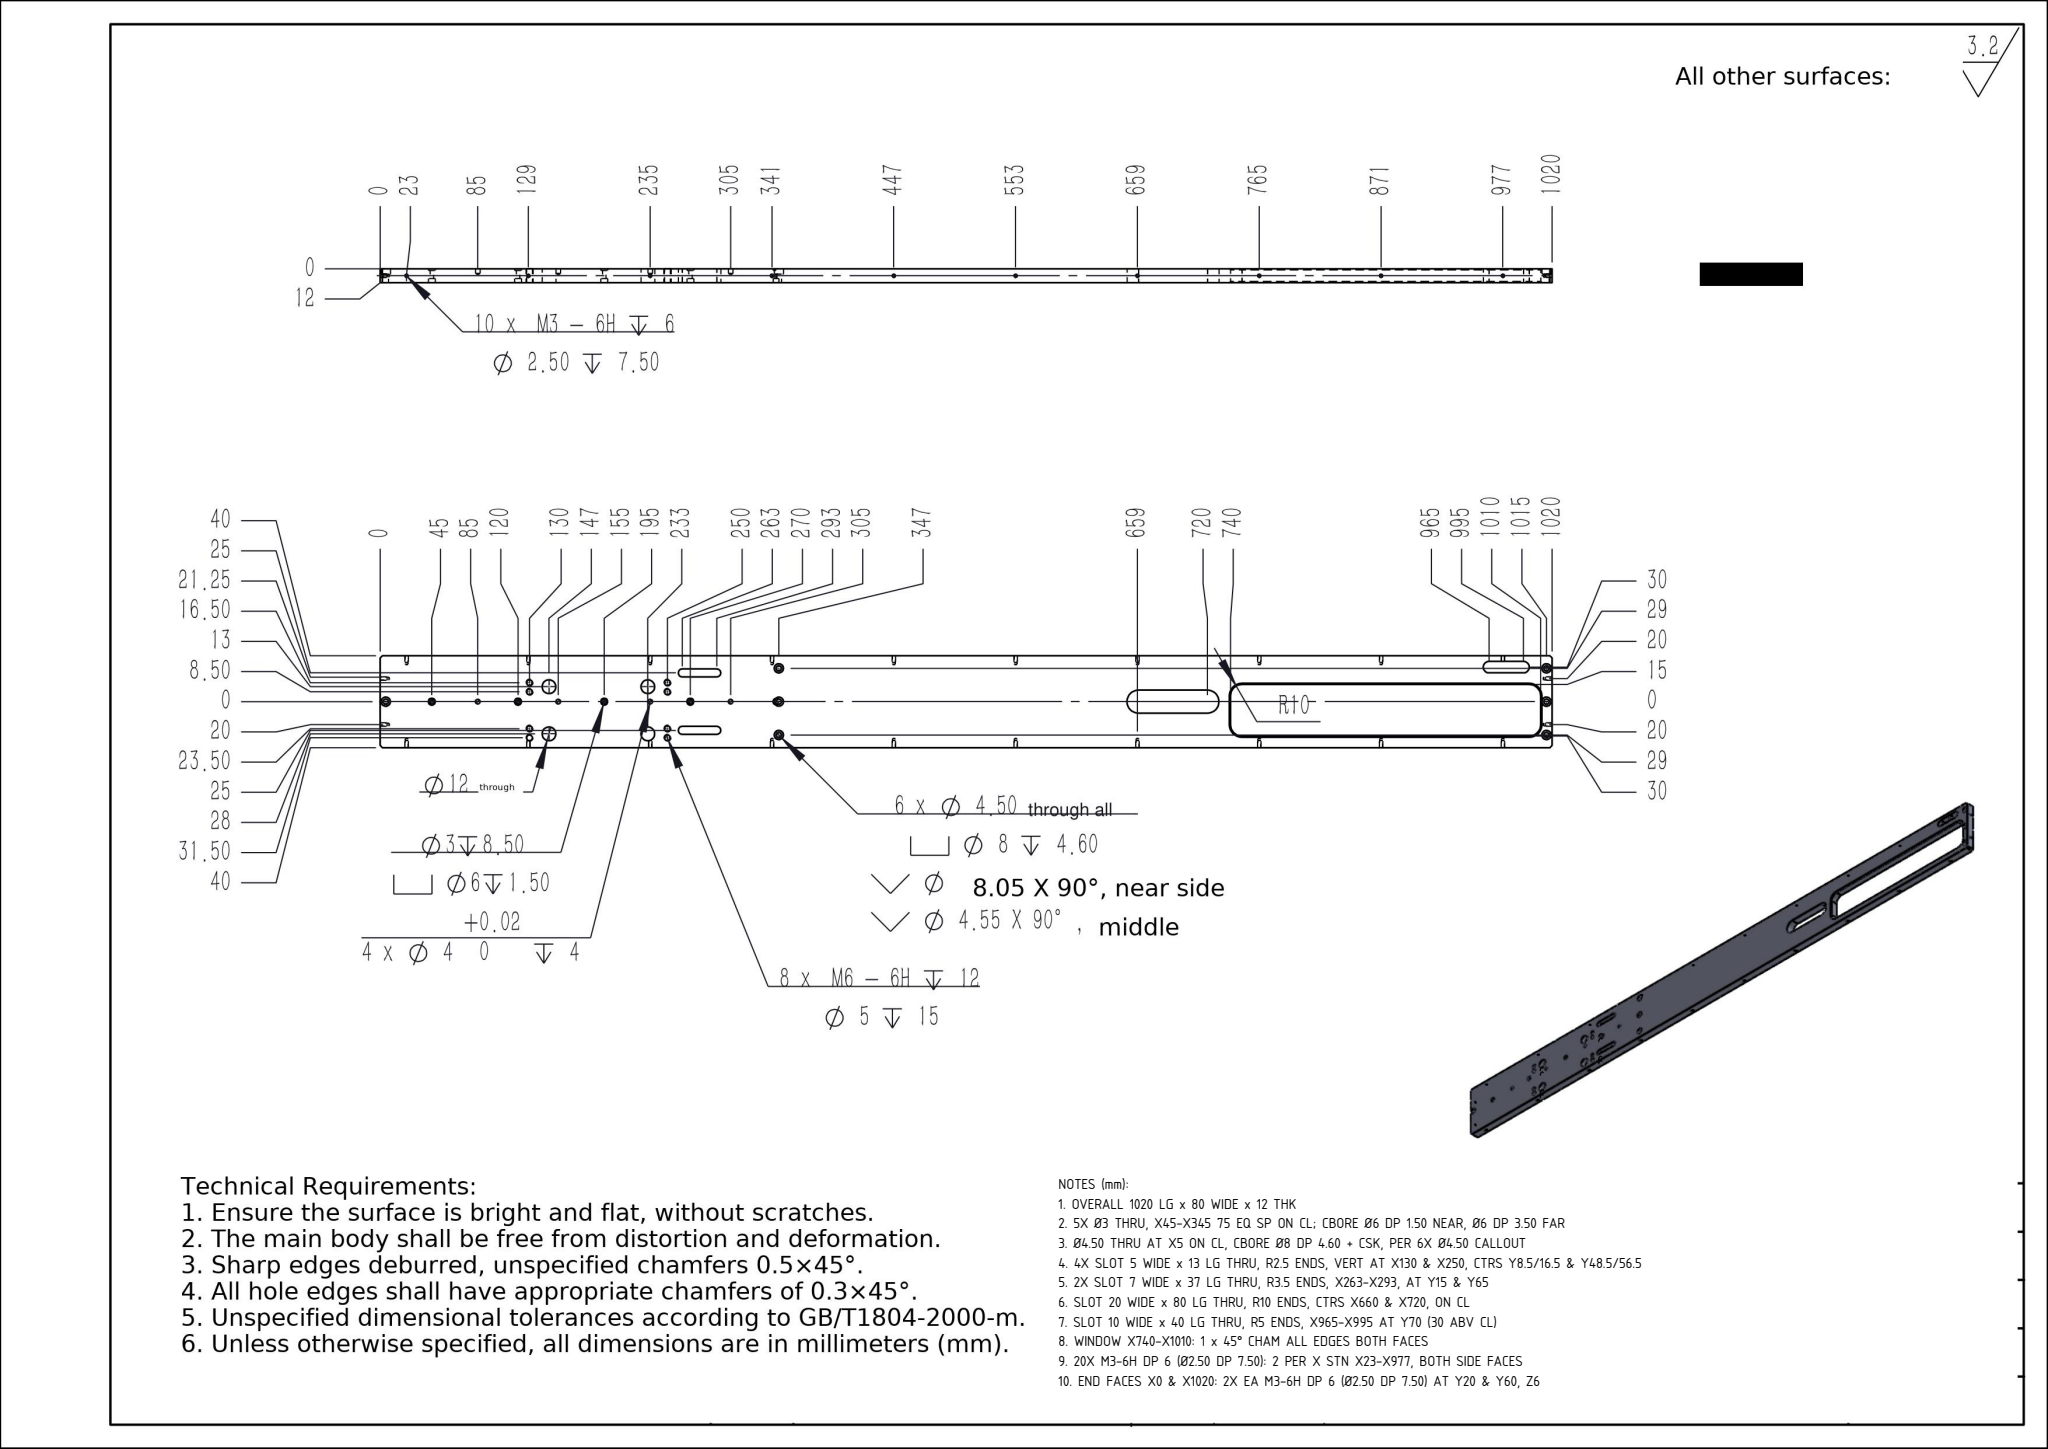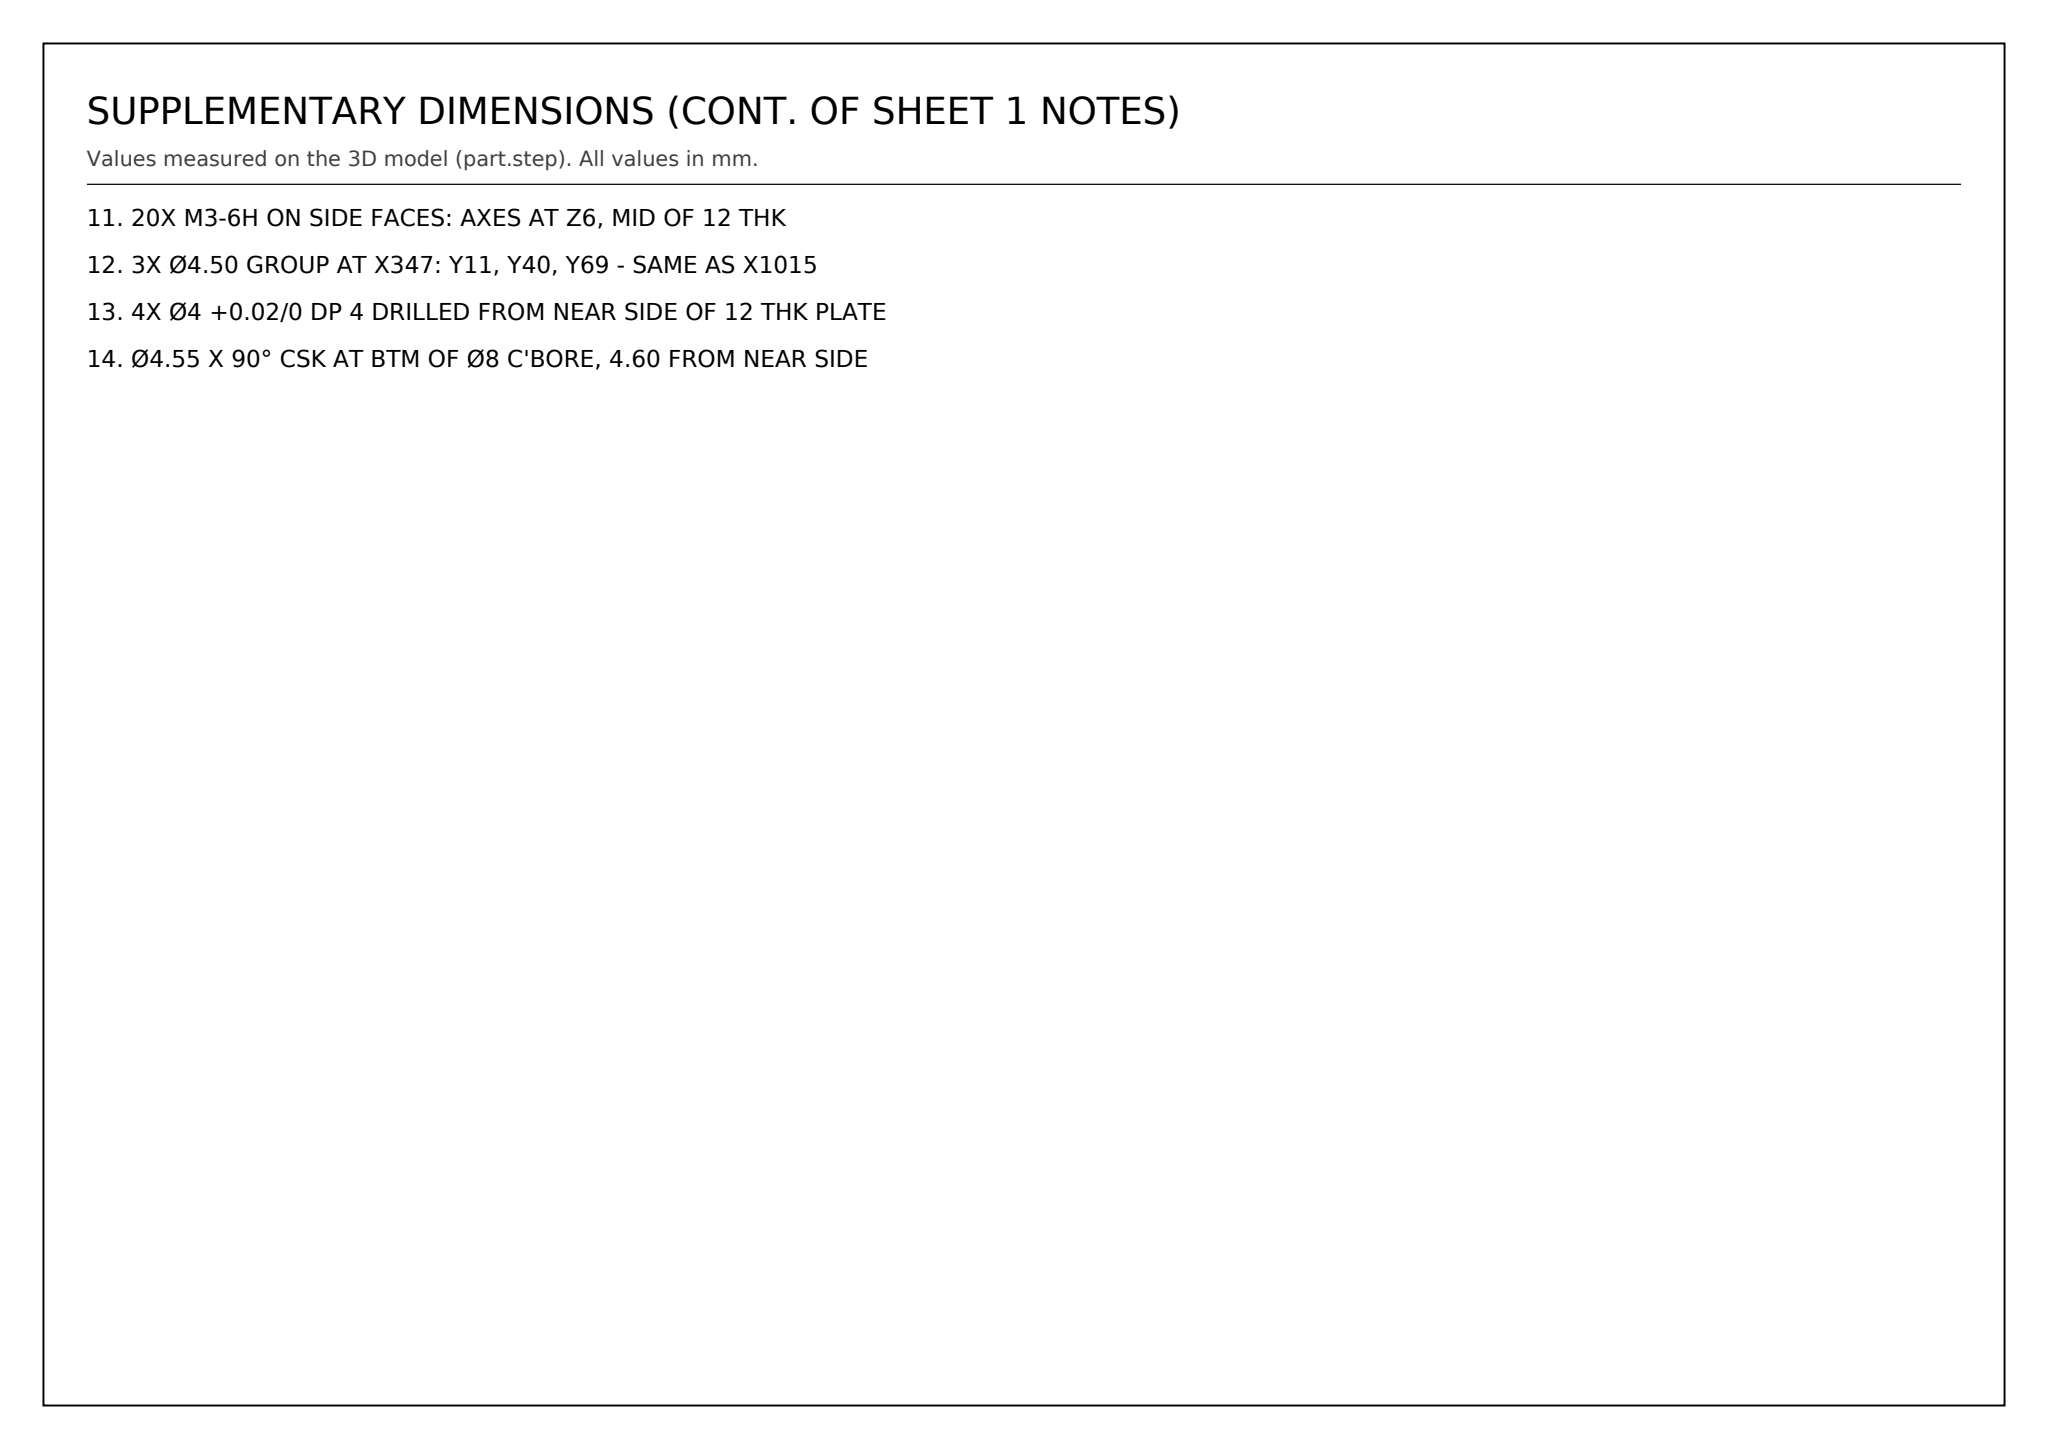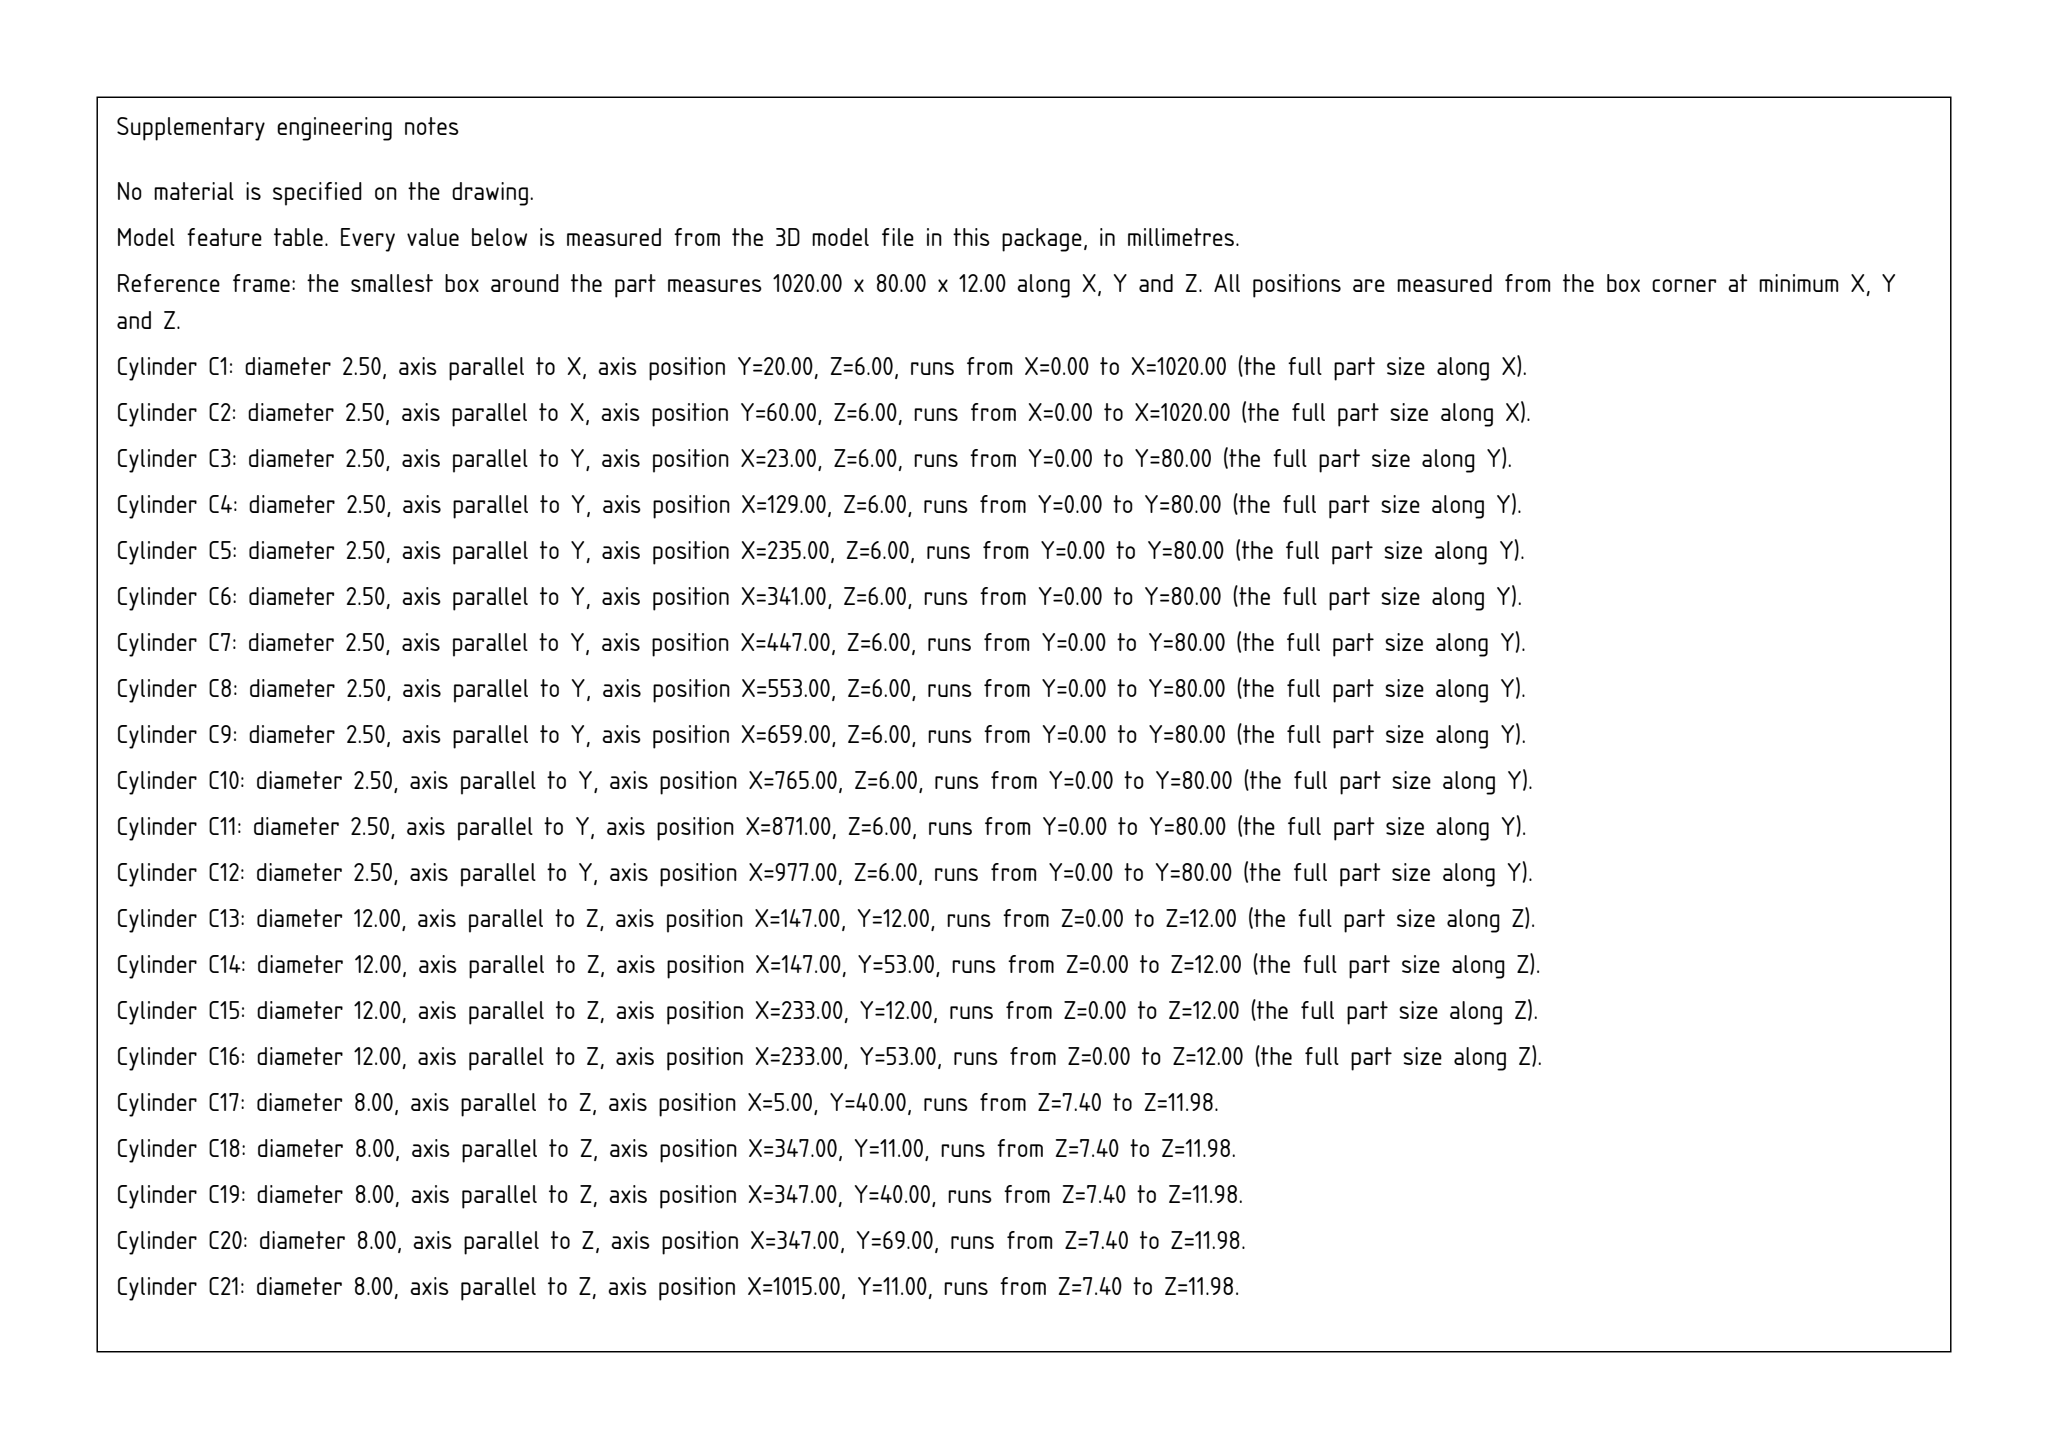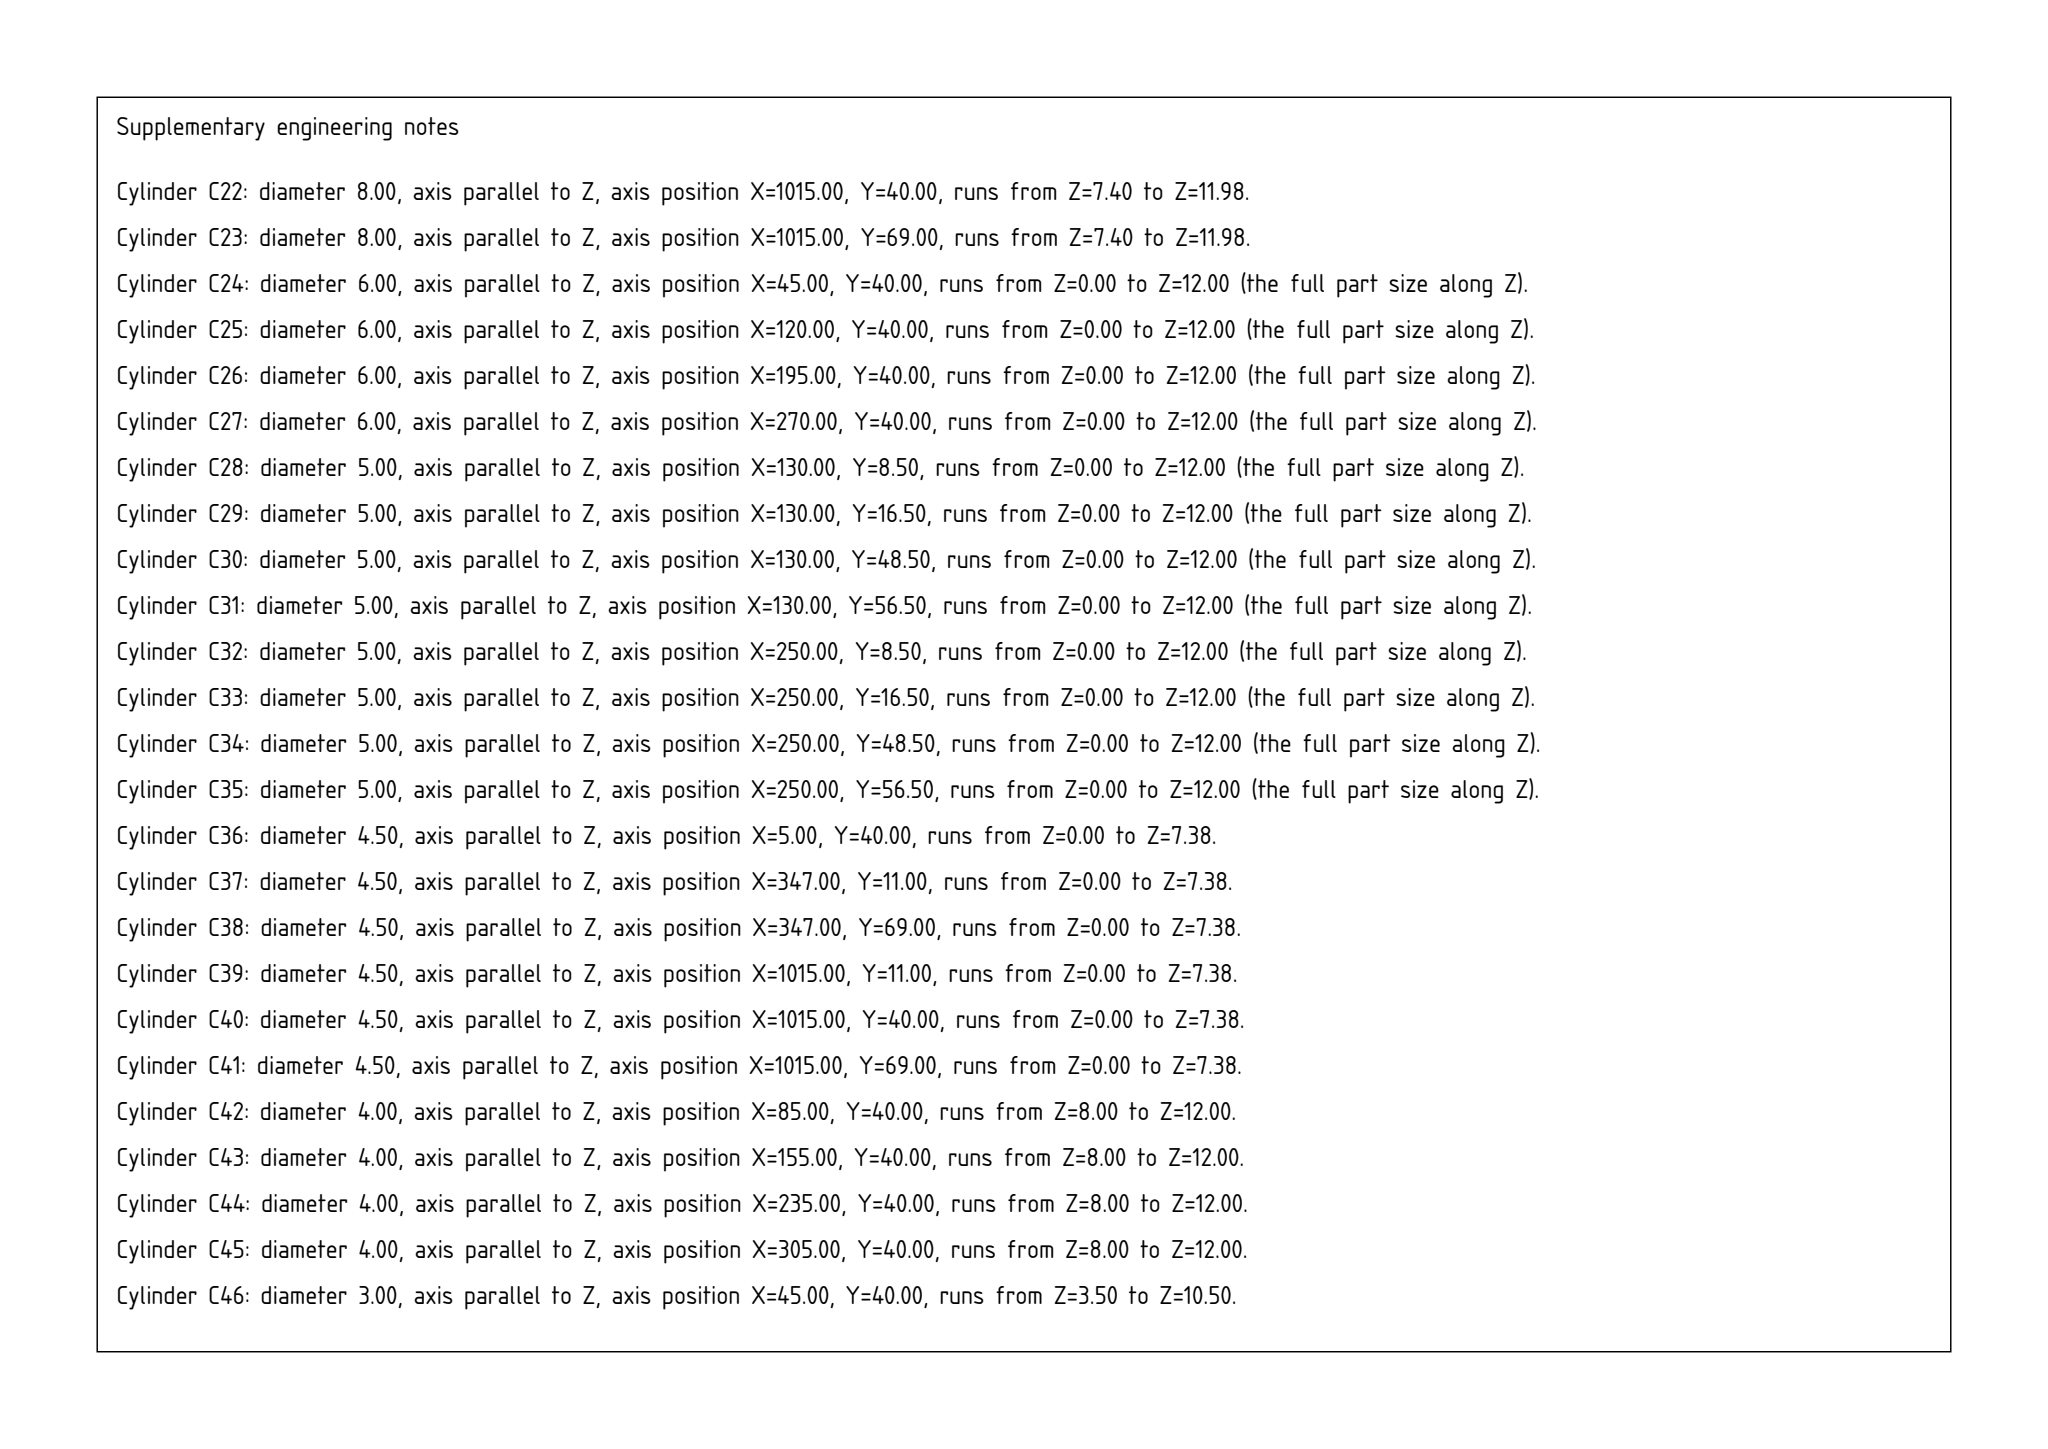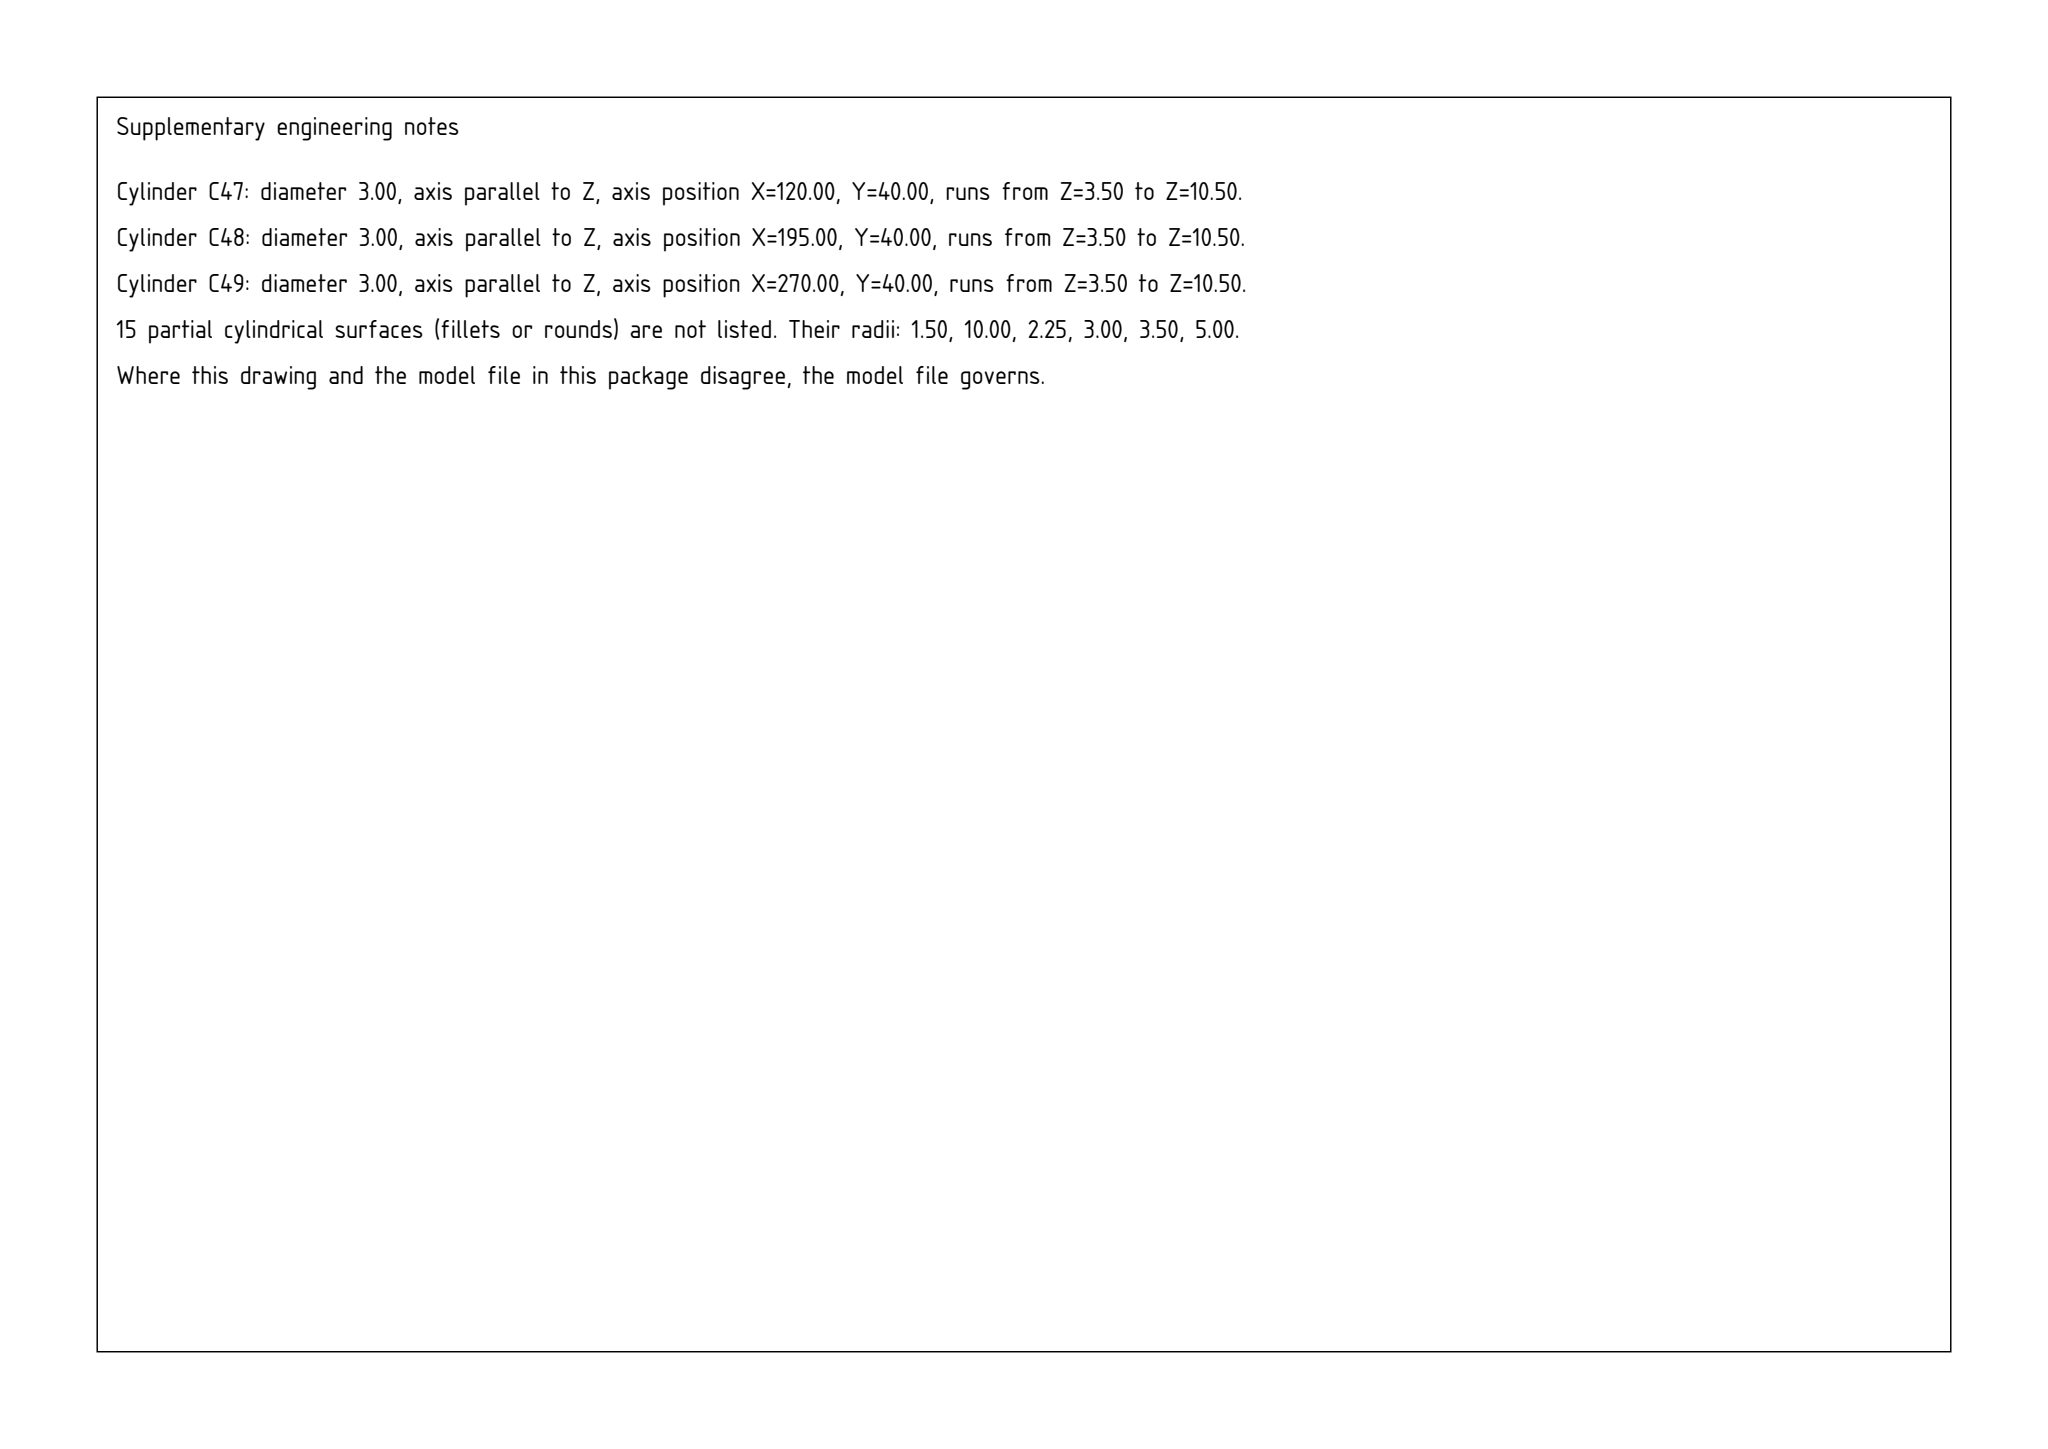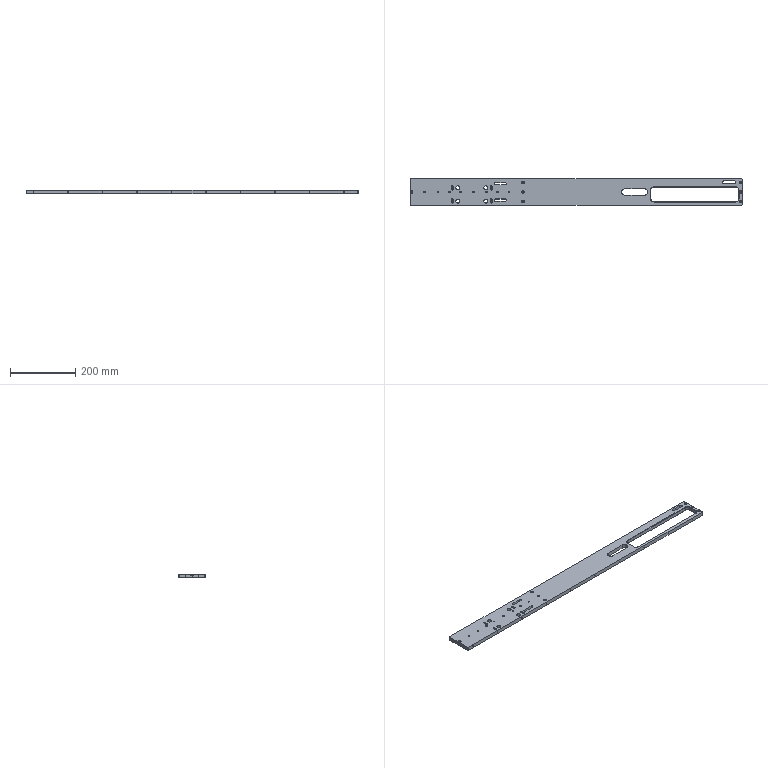Part | SolidWorks | mm | 1 solid | 285 faces | box 1020 x 80 x 12 mm | volume 793336 mm3 | cylinder 152 | cone 86 | plane 47 | commonest cylinder face diameters 2.5 x48 6 x19 5 x16 8 x14 4.5 x14 3 x9 4 x8 12 x8
Drawing notes:
OVERALL 1020 LG x 80 WIDE x 12 THK | from the solid: bbox_xyz 1020 x 80 x 12
5X Ø3 THRU, X45-X345 75 EQ SP ON CL; CBORE Ø6 DP 1.50 NEAR, Ø6 DP 3.50 FAR | from the solid: Ø3 z-cyls at X45,120,195,270,345 Y40, len 7.0; Ø6 cbores len 1.5 + 3.5 (1.5+7+3.5=12 thk)
Ø4.50 THRU AT X5 ON CL, CBORE Ø8 DP 4.60 + CSK, PER 6X Ø4.50 CALLOUT | from the solid: Ø4.5 z-cyl [5,40] len 7.38 + Ø8 cbore 4.58 + 90° cones ref 8.05/4.55
4X SLOT 5 WIDE x 13 LG THRU, R2.5 ENDS, VERT AT X130 & X250, CTRS Y8.5/16.5 & Y48.5/56.5 | from the solid: Ø5 z-cyls thru 12 at X130 & X250, Y8.5,16.5,48.5,56.5 (8 ctr-ctr = 13 LG, R2.5)
2X SLOT 7 WIDE x 37 LG THRU, R3.5 ENDS, X263-X293, AT Y15 & Y65 | from the solid: Ø7 z-cyls thru 12 at X263 & X293, Y15 and Y65 (30 ctr-ctr, R3.5 ends)
SLOT 20 WIDE x 80 LG THRU, R10 ENDS, CTRS X660 & X720, ON CL | from the solid: Ø20 z-cyls [660,40] & [720,40] len 12 thru, 60 ctr-ctr, CL y=40
SLOT 10 WIDE x 40 LG THRU, R5 ENDS, X965-X995 AT Y70 (30 ABV CL) | from the solid: Ø10 z-cyls [965,70] & [995,70] thru 12, 30 ctr-ctr, R5; y=70 = CL40 +30
WINDOW X740-X1010: 1 x 45° CHAM ALL EDGES BOTH FACES | from the solid: 90° cones ref_dia 22.0, qty 8 at R10 window corners (R10+1), 4 corners x 2 faces
20X M3-6H DP 6 (Ø2.50 DP 7.50): 2 PER X STN X23-X977, BOTH SIDE FACES | from the solid: Ø2.5 y-axis cyls at X23,129,235,341,447,553,659,765,871,977, Z6, breaking Y0 and Y80
END FACES X0 & X1020: 2X EA M3-6H DP 6 (Ø2.50 DP 7.50) AT Y20 & Y60, Z6 | from the solid: Ø2.5 x-axis cyls [null,20,6] & [null,60,6] len 7.5; planes x=0 and x=1020
20X M3-6H ON SIDE FACES: AXES AT Z6, MID OF 12 THK | from the solid: cylinders dia 2.5 axis x at z=6.0 (y=20,60) and axis y at z=6.0, plate thk 12 (z planes 0 and 12)
3X Ø4.50 GROUP AT X347: Y11, Y40, Y69 - SAME AS X1015 | from the solid: dia 4.5 axis z at [347,11],[347,40],[347,69] matching [1015,11],[1015,40],[1015,69]
4X Ø4 +0.02/0 DP 4 DRILLED FROM NEAR SIDE OF 12 THK PLATE | from the solid: Ø4 z-axis cyls at x=85,155,235,305 y=40, len 4.0 w/ 118° pt (cone 118/ref4, 8 off); 12 THK plate z0-12, near side = z12 face (Ø6 c'bore btm z=10.5, Ø8 c'bore btm z=7.4)
Ø4.55 X 90° CSK AT BTM OF Ø8 C'BORE, 4.60 FROM NEAR SIDE | from the solid: Ø8 z-cyl len 4.58 from z=12 -> plane z=7.4 (7 off, matches 7 Ø4.5 holes at 5/40, 347/11,40,69, 1015/11,40,69); Ø4.5 len 7.38 continues to z=0; 90° cone ref 4.55 at that junction